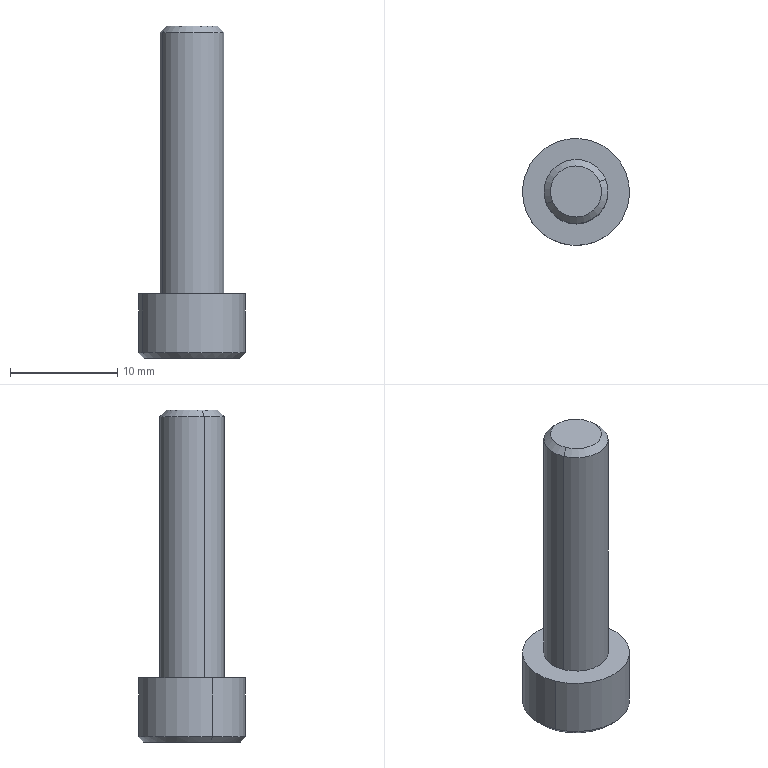Component | SolidWorks | ScrewTAC21-M6-L25(YIHEDA)-5 | 1 solid | 25 faces | box 10 x 10 x 31 mm | volume 1097 mm3 | plane 15 | cone 6 | cylinder 4 | commonest cylinder face diameters 10 x2 6 x2
STEP:
#1=COLOUR_RGB('',0.7922,0.8196,0.9333);
#2=FILL_AREA_STYLE_COLOUR('',#1);
#3=FILL_AREA_STYLE('',(#2));
#4=SURFACE_STYLE_FILL_AREA(#3);
#5=SURFACE_SIDE_STYLE('',(#4));
#6=SURFACE_STYLE_USAGE(.BOTH.,#5);
#7=PRESENTATION_STYLE_ASSIGNMENT((#6));
#8=CARTESIAN_POINT('',(0.3955,1.405,2.949));
#9=VERTEX_POINT('',#8);
#10=CARTESIAN_POINT('',(0.2219,1.333,2.949));
#11=VERTEX_POINT('',#10);
#12=CARTESIAN_POINT('',(0.3087,1.369,2.949));
#13=DIRECTION('',(0.,0.,1.));
#14=DIRECTION('',(0.9237,0.383,0.));
#15=AXIS2_PLACEMENT_3D('',#12,#13,#14);
#16=CIRCLE('',#15,0.09396);
#17=EDGE_CURVE('',#9,#11,#16,.T.);
#18=ORIENTED_EDGE('',*,*,#17,.F.);
#19=CARTESIAN_POINT('',(0.4178,1.414,2.925));
#20=VERTEX_POINT('',#19);
#21=CARTESIAN_POINT('',(0.4178,1.414,2.925));
#22=DIRECTION('',(0.6532,0.2709,-0.7071));
#23=VECTOR('',#22,39.37);
#24=LINE('',#21,#23);
#25=EDGE_CURVE('',#9,#20,#24,.T.);
#26=ORIENTED_EDGE('',*,*,#25,.T.);
#27=CARTESIAN_POINT('',(0.1996,1.323,2.925));
#28=VERTEX_POINT('',#27);
#29=CARTESIAN_POINT('',(0.3087,1.369,2.925));
#30=DIRECTION('',(0.,0.,1.));
#31=DIRECTION('',(0.9237,0.383,0.));
#32=AXIS2_PLACEMENT_3D('',#29,#30,#31);
#33=CIRCLE('',#32,0.1181);
#34=EDGE_CURVE('',#20,#28,#33,.T.);
#35=ORIENTED_EDGE('',*,*,#34,.T.);
#36=CARTESIAN_POINT('',(0.1996,1.323,2.925));
#37=DIRECTION('',(-0.6532,-0.2709,-0.7071));
#38=VECTOR('',#37,39.37);
#39=LINE('',#36,#38);
#40=EDGE_CURVE('',#11,#28,#39,.T.);
#41=ORIENTED_EDGE('',*,*,#40,.F.);
#42=EDGE_LOOP('',(#18,#26,#35,#41));
#43=FACE_OUTER_BOUND('',#42,.T.);
#44=CARTESIAN_POINT('',(0.3087,1.369,2.925));
#45=DIRECTION('',(0.,0.,-1.));
#46=DIRECTION('',(-0.9237,-0.383,0.));
#47=AXIS2_PLACEMENT_3D('',#44,#45,#46);
#48=CONICAL_SURFACE('',#47,0.1181,0.7854);
#49=ADVANCED_FACE('',(#43),#48,.T.);
#50=CARTESIAN_POINT('',(0.4723,1.437,1.728));
#51=VERTEX_POINT('',#50);
#52=CARTESIAN_POINT('',(0.145,1.301,1.728));
#53=VERTEX_POINT('',#52);
#54=CARTESIAN_POINT('',(0.3087,1.369,1.728));
#55=DIRECTION('',(0.,0.,1.));
#56=DIRECTION('',(0.9237,0.383,0.));
#57=AXIS2_PLACEMENT_3D('',#54,#55,#56);
#58=CIRCLE('',#57,0.1772);
#59=EDGE_CURVE('',#51,#53,#58,.T.);
#60=ORIENTED_EDGE('',*,*,#59,.T.);
#61=CARTESIAN_POINT('',(0.1268,1.293,1.748));
#62=VERTEX_POINT('',#61);
#63=CARTESIAN_POINT('',(0.145,1.301,1.728));
#64=DIRECTION('',(-0.6532,-0.2709,0.7071));
#65=VECTOR('',#64,39.37);
#66=LINE('',#63,#65);
#67=EDGE_CURVE('',#53,#62,#66,.T.);
#68=ORIENTED_EDGE('',*,*,#67,.T.);
#69=CARTESIAN_POINT('',(0.4905,1.444,1.748));
#70=VERTEX_POINT('',#69);
#71=CARTESIAN_POINT('',(0.3087,1.369,1.748));
#72=DIRECTION('',(0.,0.,1.));
#73=DIRECTION('',(0.9237,0.383,0.));
#74=AXIS2_PLACEMENT_3D('',#71,#72,#73);
#75=CIRCLE('',#74,0.1969);
#76=EDGE_CURVE('',#70,#62,#75,.T.);
#77=ORIENTED_EDGE('',*,*,#76,.F.);
#78=CARTESIAN_POINT('',(0.4723,1.437,1.728));
#79=DIRECTION('',(0.6532,0.2709,0.7071));
#80=VECTOR('',#79,39.37);
#81=LINE('',#78,#80);
#82=EDGE_CURVE('',#51,#70,#81,.T.);
#83=ORIENTED_EDGE('',*,*,#82,.F.);
#84=EDGE_LOOP('',(#60,#68,#77,#83));
#85=FACE_OUTER_BOUND('',#84,.T.);
#86=CARTESIAN_POINT('',(0.3087,1.369,1.728));
#87=DIRECTION('',(0.,0.,1.));
#88=DIRECTION('',(0.9237,0.383,0.));
#89=AXIS2_PLACEMENT_3D('',#86,#87,#88);
#90=CONICAL_SURFACE('',#89,0.1772,0.7854);
#91=ADVANCED_FACE('',(#85),#90,.T.);
#92=CARTESIAN_POINT('',(0.1268,1.293,1.965));
#93=VERTEX_POINT('',#92);
#94=CARTESIAN_POINT('',(0.4905,1.444,1.965));
#95=VERTEX_POINT('',#94);
#96=CARTESIAN_POINT('',(0.3087,1.369,1.965));
#97=DIRECTION('',(0.,0.,1.));
#98=DIRECTION('',(0.9237,0.383,0.));
#99=AXIS2_PLACEMENT_3D('',#96,#97,#98);
#100=CIRCLE('',#99,0.1969);
#101=EDGE_CURVE('',#93,#95,#100,.T.);
#102=ORIENTED_EDGE('',*,*,#101,.F.);
#103=CARTESIAN_POINT('',(0.1268,1.293,1.965));
#104=DIRECTION('',(0.,0.,-1.));
#105=VECTOR('',#104,39.37);
#106=LINE('',#103,#105);
#107=EDGE_CURVE('',#93,#62,#106,.T.);
#108=ORIENTED_EDGE('',*,*,#107,.T.);
#109=CARTESIAN_POINT('',(0.3087,1.369,1.748));
#110=DIRECTION('',(0.,0.,1.));
#111=DIRECTION('',(0.9237,0.383,0.));
#112=AXIS2_PLACEMENT_3D('',#109,#110,#111);
#113=CIRCLE('',#112,0.1969);
#114=EDGE_CURVE('',#62,#70,#113,.T.);
#115=ORIENTED_EDGE('',*,*,#114,.T.);
#116=CARTESIAN_POINT('',(0.4905,1.444,1.965));
#117=DIRECTION('',(0.,0.,-1.));
#118=VECTOR('',#117,39.37);
#119=LINE('',#116,#118);
#120=EDGE_CURVE('',#95,#70,#119,.T.);
#121=ORIENTED_EDGE('',*,*,#120,.F.);
#122=EDGE_LOOP('',(#102,#108,#115,#121));
#123=FACE_OUTER_BOUND('',#122,.T.);
#124=CARTESIAN_POINT('',(0.3087,1.369,1.965));
#125=DIRECTION('',(0.,0.,-1.));
#126=DIRECTION('',(0.9237,0.383,0.));
#127=AXIS2_PLACEMENT_3D('',#124,#125,#126);
#128=CYLINDRICAL_SURFACE('',#127,0.1969);
#129=ADVANCED_FACE('',(#123),#128,.T.);
#130=CARTESIAN_POINT('',(0.3087,1.369,1.903));
#131=VERTEX_POINT('',#130);
#132=CARTESIAN_POINT('',(0.2178,1.331,1.847));
#133=VERTEX_POINT('',#132);
#134=CARTESIAN_POINT('',(0.2178,1.331,1.847));
#135=DIRECTION('',(-0.8,-0.3317,-0.5));
#136=VECTOR('',#135,39.37);
#137=LINE('',#134,#136);
#138=EDGE_CURVE('',#131,#133,#137,.T.);
#139=ORIENTED_EDGE('',*,*,#138,.F.);
#140=CARTESIAN_POINT('',(0.3996,1.406,1.847));
#141=VERTEX_POINT('',#140);
#142=CARTESIAN_POINT('',(0.3996,1.406,1.847));
#143=DIRECTION('',(0.8,0.3317,-0.5));
#144=VECTOR('',#143,39.37);
#145=LINE('',#142,#144);
#146=EDGE_CURVE('',#131,#141,#145,.T.);
#147=ORIENTED_EDGE('',*,*,#146,.T.);
#148=CARTESIAN_POINT('',(0.3868,1.309,1.847));
#149=VERTEX_POINT('',#148);
#150=CARTESIAN_POINT('',(0.3087,1.369,1.847));
#151=DIRECTION('',(0.,0.,1.));
#152=DIRECTION('',(-0.9237,-0.383,0.));
#153=AXIS2_PLACEMENT_3D('',#150,#151,#152);
#154=CIRCLE('',#153,0.09843);
#155=EDGE_CURVE('',#149,#141,#154,.T.);
#156=ORIENTED_EDGE('',*,*,#155,.F.);
#157=CARTESIAN_POINT('',(0.2959,1.271,1.847));
#158=VERTEX_POINT('',#157);
#159=CARTESIAN_POINT('',(0.3087,1.369,1.847));
#160=DIRECTION('',(0.,0.,1.));
#161=DIRECTION('',(-0.9237,-0.383,0.));
#162=AXIS2_PLACEMENT_3D('',#159,#160,#161);
#163=CIRCLE('',#162,0.09843);
#164=EDGE_CURVE('',#158,#149,#163,.T.);
#165=ORIENTED_EDGE('',*,*,#164,.F.);
#166=CARTESIAN_POINT('',(0.3087,1.369,1.847));
#167=DIRECTION('',(0.,0.,1.));
#168=DIRECTION('',(-0.9237,-0.383,0.));
#169=AXIS2_PLACEMENT_3D('',#166,#167,#168);
#170=CIRCLE('',#169,0.09843);
#171=EDGE_CURVE('',#133,#158,#170,.T.);
#172=ORIENTED_EDGE('',*,*,#171,.F.);
#173=EDGE_LOOP('',(#139,#147,#156,#165,#172));
#174=FACE_OUTER_BOUND('',#173,.T.);
#175=CARTESIAN_POINT('',(0.3087,1.369,1.847));
#176=DIRECTION('',(0.,0.,-1.));
#177=DIRECTION('',(-0.9237,-0.383,0.));
#178=AXIS2_PLACEMENT_3D('',#175,#176,#177);
#179=CONICAL_SURFACE('',#178,0.09843,1.047);
#180=ADVANCED_FACE('',(#174),#179,.F.);
#181=CARTESIAN_POINT('',(0.3087,1.369,2.925));
#182=DIRECTION('',(0.,0.,1.));
#183=DIRECTION('',(0.9237,0.383,0.));
#184=AXIS2_PLACEMENT_3D('',#181,#182,#183);
#185=CIRCLE('',#184,0.1181);
#186=EDGE_CURVE('',#28,#20,#185,.T.);
#187=ORIENTED_EDGE('',*,*,#186,.F.);
#188=CARTESIAN_POINT('',(0.1996,1.323,1.965));
#189=VERTEX_POINT('',#188);
#190=CARTESIAN_POINT('',(0.1996,1.323,2.949));
#191=DIRECTION('',(0.,0.,-1.));
#192=VECTOR('',#191,39.37);
#193=LINE('',#190,#192);
#194=EDGE_CURVE('',#28,#189,#193,.T.);
#195=ORIENTED_EDGE('',*,*,#194,.T.);
#196=CARTESIAN_POINT('',(0.4178,1.414,1.965));
#197=VERTEX_POINT('',#196);
#198=CARTESIAN_POINT('',(0.3087,1.369,1.965));
#199=DIRECTION('',(0.,0.,1.));
#200=DIRECTION('',(0.9237,0.383,0.));
#201=AXIS2_PLACEMENT_3D('',#198,#199,#200);
#202=CIRCLE('',#201,0.1181);
#203=EDGE_CURVE('',#189,#197,#202,.T.);
#204=ORIENTED_EDGE('',*,*,#203,.T.);
#205=CARTESIAN_POINT('',(0.4178,1.414,2.949));
#206=DIRECTION('',(0.,0.,-1.));
#207=VECTOR('',#206,39.37);
#208=LINE('',#205,#207);
#209=EDGE_CURVE('',#20,#197,#208,.T.);
#210=ORIENTED_EDGE('',*,*,#209,.F.);
#211=EDGE_LOOP('',(#187,#195,#204,#210));
#212=FACE_OUTER_BOUND('',#211,.T.);
#213=CARTESIAN_POINT('',(0.3087,1.369,2.949));
#214=DIRECTION('',(0.,0.,-1.));
#215=DIRECTION('',(0.9237,0.383,0.));
#216=AXIS2_PLACEMENT_3D('',#213,#214,#215);
#217=CYLINDRICAL_SURFACE('',#216,0.1181);
#218=ADVANCED_FACE('',(#212),#217,.T.);
#219=CARTESIAN_POINT('',(0.3522,1.264,1.847));
#220=VERTEX_POINT('',#219);
#221=CARTESIAN_POINT('',(0.3522,1.264,1.847));
#222=DIRECTION('',(-0.9915,0.1301,0.));
#223=VECTOR('',#222,39.37);
#224=LINE('',#221,#223);
#225=EDGE_CURVE('',#220,#158,#224,.T.);
#226=ORIENTED_EDGE('',*,*,#225,.T.);
#227=ORIENTED_EDGE('',*,*,#164,.T.);
#228=CARTESIAN_POINT('',(0.4214,1.354,1.847));
#229=DIRECTION('',(-0.6084,-0.7936,0.));
#230=VECTOR('',#229,39.37);
#231=LINE('',#228,#230);
#232=EDGE_CURVE('',#149,#220,#231,.T.);
#233=ORIENTED_EDGE('',*,*,#232,.T.);
#234=EDGE_LOOP('',(#226,#227,#233));
#235=FACE_OUTER_BOUND('',#234,.T.);
#236=CARTESIAN_POINT('',(0.3087,1.369,1.847));
#237=DIRECTION('',(0.,0.,-1.));
#238=DIRECTION('',(-0.9237,-0.383,0.));
#239=AXIS2_PLACEMENT_3D('',#236,#237,#238);
#240=PLANE('',#239);
#241=ADVANCED_FACE('',(#235),#240,.T.);
#242=ORIENTED_EDGE('',*,*,#194,.F.);
#243=ORIENTED_EDGE('',*,*,#34,.F.);
#244=ORIENTED_EDGE('',*,*,#209,.T.);
#245=CARTESIAN_POINT('',(0.3087,1.369,1.965));
#246=DIRECTION('',(0.,0.,1.));
#247=DIRECTION('',(0.9237,0.383,0.));
#248=AXIS2_PLACEMENT_3D('',#245,#246,#247);
#249=CIRCLE('',#248,0.1181);
#250=EDGE_CURVE('',#197,#189,#249,.T.);
#251=ORIENTED_EDGE('',*,*,#250,.T.);
#252=EDGE_LOOP('',(#242,#243,#244,#251));
#253=FACE_OUTER_BOUND('',#252,.T.);
#254=CARTESIAN_POINT('',(0.3087,1.369,2.949));
#255=DIRECTION('',(0.,0.,-1.));
#256=DIRECTION('',(0.9237,0.383,0.));
#257=AXIS2_PLACEMENT_3D('',#254,#255,#256);
#258=CYLINDRICAL_SURFACE('',#257,0.1181);
#259=ADVANCED_FACE('',(#253),#258,.T.);
#260=ORIENTED_EDGE('',*,*,#146,.F.);
#261=ORIENTED_EDGE('',*,*,#138,.T.);
#262=CARTESIAN_POINT('',(0.2306,1.429,1.847));
#263=VERTEX_POINT('',#262);
#264=CARTESIAN_POINT('',(0.3087,1.369,1.847));
#265=DIRECTION('',(0.,0.,1.));
#266=DIRECTION('',(-0.9237,-0.383,0.));
#267=AXIS2_PLACEMENT_3D('',#264,#265,#266);
#268=CIRCLE('',#267,0.09843);
#269=EDGE_CURVE('',#263,#133,#268,.T.);
#270=ORIENTED_EDGE('',*,*,#269,.F.);
#271=CARTESIAN_POINT('',(0.3215,1.466,1.847));
#272=VERTEX_POINT('',#271);
#273=CARTESIAN_POINT('',(0.3087,1.369,1.847));
#274=DIRECTION('',(0.,0.,1.));
#275=DIRECTION('',(-0.9237,-0.383,0.));
#276=AXIS2_PLACEMENT_3D('',#273,#274,#275);
#277=CIRCLE('',#276,0.09843);
#278=EDGE_CURVE('',#272,#263,#277,.T.);
#279=ORIENTED_EDGE('',*,*,#278,.F.);
#280=CARTESIAN_POINT('',(0.3087,1.369,1.847));
#281=DIRECTION('',(0.,0.,1.));
#282=DIRECTION('',(-0.9237,-0.383,0.));
#283=AXIS2_PLACEMENT_3D('',#280,#281,#282);
#284=CIRCLE('',#283,0.09843);
#285=EDGE_CURVE('',#141,#272,#284,.T.);
#286=ORIENTED_EDGE('',*,*,#285,.F.);
#287=EDGE_LOOP('',(#260,#261,#270,#279,#286));
#288=FACE_OUTER_BOUND('',#287,.T.);
#289=CARTESIAN_POINT('',(0.3087,1.369,1.847));
#290=DIRECTION('',(0.,0.,-1.));
#291=DIRECTION('',(-0.9237,-0.383,0.));
#292=AXIS2_PLACEMENT_3D('',#289,#290,#291);
#293=CONICAL_SURFACE('',#292,0.09843,1.047);
#294=ADVANCED_FACE('',(#288),#293,.F.);
#295=CARTESIAN_POINT('',(0.3778,1.459,1.728));
#296=VERTEX_POINT('',#295);
#297=CARTESIAN_POINT('',(0.4214,1.354,1.728));
#298=VERTEX_POINT('',#297);
#299=CARTESIAN_POINT('',(0.3778,1.459,1.728));
#300=DIRECTION('',(0.383,-0.9237,0.));
#301=VECTOR('',#300,39.37);
#302=LINE('',#299,#301);
#303=EDGE_CURVE('',#296,#298,#302,.T.);
#304=ORIENTED_EDGE('',*,*,#303,.T.);
#305=CARTESIAN_POINT('',(0.4214,1.354,1.847));
#306=VERTEX_POINT('',#305);
#307=CARTESIAN_POINT('',(0.4214,1.354,1.847));
#308=DIRECTION('',(0.,0.,-1.));
#309=VECTOR('',#308,39.37);
#310=LINE('',#307,#309);
#311=EDGE_CURVE('',#306,#298,#310,.T.);
#312=ORIENTED_EDGE('',*,*,#311,.F.);
#313=CARTESIAN_POINT('',(0.3778,1.459,1.847));
#314=DIRECTION('',(0.383,-0.9237,0.));
#315=VECTOR('',#314,39.37);
#316=LINE('',#313,#315);
#317=EDGE_CURVE('',#141,#306,#316,.T.);
#318=ORIENTED_EDGE('',*,*,#317,.F.);
#319=CARTESIAN_POINT('',(0.3778,1.459,1.847));
#320=VERTEX_POINT('',#319);
#321=CARTESIAN_POINT('',(0.3778,1.459,1.847));
#322=DIRECTION('',(0.383,-0.9237,0.));
#323=VECTOR('',#322,39.37);
#324=LINE('',#321,#323);
#325=EDGE_CURVE('',#320,#141,#324,.T.);
#326=ORIENTED_EDGE('',*,*,#325,.F.);
#327=CARTESIAN_POINT('',(0.3778,1.459,1.847));
#328=DIRECTION('',(0.,0.,-1.));
#329=VECTOR('',#328,39.37);
#330=LINE('',#327,#329);
#331=EDGE_CURVE('',#320,#296,#330,.T.);
#332=ORIENTED_EDGE('',*,*,#331,.T.);
#333=EDGE_LOOP('',(#304,#312,#318,#326,#332));
#334=FACE_OUTER_BOUND('',#333,.T.);
#335=CARTESIAN_POINT('',(0.3778,1.459,1.847));
#336=DIRECTION('',(0.9237,0.383,0.));
#337=DIRECTION('',(0.,0.,-1.));
#338=AXIS2_PLACEMENT_3D('',#335,#336,#337);
#339=PLANE('',#338);
#340=ADVANCED_FACE('',(#334),#339,.F.);
#341=CARTESIAN_POINT('',(0.196,1.384,1.728));
#342=VERTEX_POINT('',#341);
#343=CARTESIAN_POINT('',(0.2651,1.474,1.728));
#344=VERTEX_POINT('',#343);
#345=CARTESIAN_POINT('',(0.196,1.384,1.728));
#346=DIRECTION('',(0.6084,0.7936,0.));
#347=VECTOR('',#346,39.37);
#348=LINE('',#345,#347);
#349=EDGE_CURVE('',#342,#344,#348,.T.);
#350=ORIENTED_EDGE('',*,*,#349,.T.);
#351=CARTESIAN_POINT('',(0.2651,1.474,1.847));
#352=VERTEX_POINT('',#351);
#353=CARTESIAN_POINT('',(0.2651,1.474,1.847));
#354=DIRECTION('',(0.,0.,-1.));
#355=VECTOR('',#354,39.37);
#356=LINE('',#353,#355);
#357=EDGE_CURVE('',#352,#344,#356,.T.);
#358=ORIENTED_EDGE('',*,*,#357,.F.);
#359=CARTESIAN_POINT('',(0.196,1.384,1.847));
#360=DIRECTION('',(0.6084,0.7936,0.));
#361=VECTOR('',#360,39.37);
#362=LINE('',#359,#361);
#363=EDGE_CURVE('',#263,#352,#362,.T.);
#364=ORIENTED_EDGE('',*,*,#363,.F.);
#365=CARTESIAN_POINT('',(0.196,1.384,1.847));
#366=VERTEX_POINT('',#365);
#367=CARTESIAN_POINT('',(0.196,1.384,1.847));
#368=DIRECTION('',(0.6084,0.7936,0.));
#369=VECTOR('',#368,39.37);
#370=LINE('',#367,#369);
#371=EDGE_CURVE('',#366,#263,#370,.T.);
#372=ORIENTED_EDGE('',*,*,#371,.F.);
#373=CARTESIAN_POINT('',(0.196,1.384,1.847));
#374=DIRECTION('',(0.,0.,-1.));
#375=VECTOR('',#374,39.37);
#376=LINE('',#373,#375);
#377=EDGE_CURVE('',#366,#342,#376,.T.);
#378=ORIENTED_EDGE('',*,*,#377,.T.);
#379=EDGE_LOOP('',(#350,#358,#364,#372,#378));
#380=FACE_OUTER_BOUND('',#379,.T.);
#381=CARTESIAN_POINT('',(0.196,1.384,1.847));
#382=DIRECTION('',(-0.7936,0.6084,0.));
#383=DIRECTION('',(0.,0.,1.));
#384=AXIS2_PLACEMENT_3D('',#381,#382,#383);
#385=PLANE('',#384);
#386=ADVANCED_FACE('',(#380),#385,.F.);
#387=ORIENTED_EDGE('',*,*,#371,.T.);
#388=ORIENTED_EDGE('',*,*,#269,.T.);
#389=CARTESIAN_POINT('',(0.2395,1.279,1.847));
#390=DIRECTION('',(-0.383,0.9237,0.));
#391=VECTOR('',#390,39.37);
#392=LINE('',#389,#391);
#393=EDGE_CURVE('',#133,#366,#392,.T.);
#394=ORIENTED_EDGE('',*,*,#393,.T.);
#395=EDGE_LOOP('',(#387,#388,#394));
#396=FACE_OUTER_BOUND('',#395,.T.);
#397=CARTESIAN_POINT('',(0.3087,1.369,1.847));
#398=DIRECTION('',(0.,0.,-1.));
#399=DIRECTION('',(-0.9237,-0.383,0.));
#400=AXIS2_PLACEMENT_3D('',#397,#398,#399);
#401=PLANE('',#400);
#402=ADVANCED_FACE('',(#396),#401,.T.);
#403=CARTESIAN_POINT('',(0.3087,1.369,1.965));
#404=DIRECTION('',(0.,0.,1.));
#405=DIRECTION('',(0.9237,0.383,0.));
#406=AXIS2_PLACEMENT_3D('',#403,#404,#405);
#407=CIRCLE('',#406,0.1969);
#408=EDGE_CURVE('',#95,#93,#407,.T.);
#409=ORIENTED_EDGE('',*,*,#408,.T.);
#410=ORIENTED_EDGE('',*,*,#101,.T.);
#411=EDGE_LOOP('',(#409,#410));
#412=FACE_OUTER_BOUND('',#411,.T.);
#413=ORIENTED_EDGE('',*,*,#250,.F.);
#414=ORIENTED_EDGE('',*,*,#203,.F.);
#415=EDGE_LOOP('',(#413,#414));
#416=FACE_BOUND('',#415,.T.);
#417=CARTESIAN_POINT('',(0.2333,1.551,1.965));
#418=DIRECTION('',(0.,0.,-1.));
#419=DIRECTION('',(-0.9237,-0.383,0.));
#420=AXIS2_PLACEMENT_3D('',#417,#418,#419);
#421=PLANE('',#420);
#422=ADVANCED_FACE('',(#412,#416),#421,.F.);
#423=ORIENTED_EDGE('',*,*,#59,.F.);
#424=CARTESIAN_POINT('',(0.3087,1.369,1.728));
#425=DIRECTION('',(0.,0.,1.));
#426=DIRECTION('',(0.9237,0.383,0.));
#427=AXIS2_PLACEMENT_3D('',#424,#425,#426);
#428=CIRCLE('',#427,0.1772);
#429=EDGE_CURVE('',#53,#51,#428,.T.);
#430=ORIENTED_EDGE('',*,*,#429,.F.);
#431=EDGE_LOOP('',(#423,#430));
#432=FACE_OUTER_BOUND('',#431,.T.);
#433=CARTESIAN_POINT('',(0.3522,1.264,1.728));
#434=VERTEX_POINT('',#433);
#435=CARTESIAN_POINT('',(0.2395,1.279,1.728));
#436=VERTEX_POINT('',#435);
#437=CARTESIAN_POINT('',(0.3522,1.264,1.728));
#438=DIRECTION('',(-0.9915,0.1301,0.));
#439=VECTOR('',#438,39.37);
#440=LINE('',#437,#439);
#441=EDGE_CURVE('',#434,#436,#440,.T.);
#442=ORIENTED_EDGE('',*,*,#441,.F.);
#443=CARTESIAN_POINT('',(0.4214,1.354,1.728));
#444=DIRECTION('',(-0.6084,-0.7936,0.));
#445=VECTOR('',#444,39.37);
#446=LINE('',#443,#445);
#447=EDGE_CURVE('',#298,#434,#446,.T.);
#448=ORIENTED_EDGE('',*,*,#447,.F.);
#449=ORIENTED_EDGE('',*,*,#303,.F.);
#450=CARTESIAN_POINT('',(0.2651,1.474,1.728));
#451=DIRECTION('',(0.9915,-0.1301,0.));
#452=VECTOR('',#451,39.37);
#453=LINE('',#450,#452);
#454=EDGE_CURVE('',#344,#296,#453,.T.);
#455=ORIENTED_EDGE('',*,*,#454,.F.);
#456=ORIENTED_EDGE('',*,*,#349,.F.);
#457=CARTESIAN_POINT('',(0.2395,1.279,1.728));
#458=DIRECTION('',(-0.383,0.9237,0.));
#459=VECTOR('',#458,39.37);
#460=LINE('',#457,#459);
#461=EDGE_CURVE('',#436,#342,#460,.T.);
#462=ORIENTED_EDGE('',*,*,#461,.F.);
#463=EDGE_LOOP('',(#442,#448,#449,#455,#456,#462));
#464=FACE_BOUND('',#463,.T.);
#465=CARTESIAN_POINT('',(0.3087,1.369,1.728));
#466=DIRECTION('',(0.,0.,1.));
#467=DIRECTION('',(0.383,-0.9237,0.));
#468=AXIS2_PLACEMENT_3D('',#465,#466,#467);
#469=PLANE('',#468);
#470=ADVANCED_FACE('',(#432,#464),#469,.F.);
#471=CARTESIAN_POINT('',(0.3087,1.369,2.949));
#472=DIRECTION('',(0.,0.,1.));
#473=DIRECTION('',(0.9237,0.383,0.));
#474=AXIS2_PLACEMENT_3D('',#471,#472,#473);
#475=CIRCLE('',#474,0.09396);
#476=EDGE_CURVE('',#11,#9,#475,.T.);
#477=ORIENTED_EDGE('',*,*,#476,.T.);
#478=ORIENTED_EDGE('',*,*,#17,.T.);
#479=EDGE_LOOP('',(#477,#478));
#480=FACE_OUTER_BOUND('',#479,.T.);
#481=CARTESIAN_POINT('',(0.2727,1.456,2.949));
#482=DIRECTION('',(0.,0.,-1.));
#483=DIRECTION('',(-0.9237,-0.383,0.));
#484=AXIS2_PLACEMENT_3D('',#481,#482,#483);
#485=PLANE('',#484);
#486=ADVANCED_FACE('',(#480),#485,.F.);
#487=ORIENTED_EDGE('',*,*,#107,.F.);
#488=ORIENTED_EDGE('',*,*,#408,.F.);
#489=ORIENTED_EDGE('',*,*,#120,.T.);
#490=ORIENTED_EDGE('',*,*,#76,.T.);
#491=EDGE_LOOP('',(#487,#488,#489,#490));
#492=FACE_OUTER_BOUND('',#491,.T.);
#493=CARTESIAN_POINT('',(0.3087,1.369,1.965));
#494=DIRECTION('',(0.,0.,-1.));
#495=DIRECTION('',(0.9237,0.383,0.));
#496=AXIS2_PLACEMENT_3D('',#493,#494,#495);
#497=CYLINDRICAL_SURFACE('',#496,0.1969);
#498=ADVANCED_FACE('',(#492),#497,.T.);
#499=ORIENTED_EDGE('',*,*,#447,.T.);
#500=CARTESIAN_POINT('',(0.3522,1.264,1.847));
#501=DIRECTION('',(0.,0.,-1.));
#502=VECTOR('',#501,39.37);
#503=LINE('',#500,#502);
#504=EDGE_CURVE('',#220,#434,#503,.T.);
#505=ORIENTED_EDGE('',*,*,#504,.F.);
#506=ORIENTED_EDGE('',*,*,#232,.F.);
#507=CARTESIAN_POINT('',(0.4214,1.354,1.847));
#508=DIRECTION('',(-0.6084,-0.7936,0.));
#509=VECTOR('',#508,39.37);
#510=LINE('',#507,#509);
#511=EDGE_CURVE('',#306,#149,#510,.T.);
#512=ORIENTED_EDGE('',*,*,#511,.F.);
#513=ORIENTED_EDGE('',*,*,#311,.T.);
#514=EDGE_LOOP('',(#499,#505,#506,#512,#513));
#515=FACE_OUTER_BOUND('',#514,.T.);
#516=CARTESIAN_POINT('',(0.4214,1.354,1.847));
#517=DIRECTION('',(0.7936,-0.6084,0.));
#518=DIRECTION('',(0.6084,0.7936,0.));
#519=AXIS2_PLACEMENT_3D('',#516,#517,#518);
#520=PLANE('',#519);
#521=ADVANCED_FACE('',(#515),#520,.F.);
#522=ORIENTED_EDGE('',*,*,#67,.F.);
#523=ORIENTED_EDGE('',*,*,#429,.T.);
#524=ORIENTED_EDGE('',*,*,#82,.T.);
#525=ORIENTED_EDGE('',*,*,#114,.F.);
#526=EDGE_LOOP('',(#522,#523,#524,#525));
#527=FACE_OUTER_BOUND('',#526,.T.);
#528=CARTESIAN_POINT('',(0.3087,1.369,1.728));
#529=DIRECTION('',(0.,0.,1.));
#530=DIRECTION('',(0.9237,0.383,0.));
#531=AXIS2_PLACEMENT_3D('',#528,#529,#530);
#532=CONICAL_SURFACE('',#531,0.1772,0.7854);
#533=ADVANCED_FACE('',(#527),#532,.T.);
#534=ORIENTED_EDGE('',*,*,#441,.T.);
#535=CARTESIAN_POINT('',(0.2395,1.279,1.847));
#536=VERTEX_POINT('',#535);
#537=CARTESIAN_POINT('',(0.2395,1.279,1.847));
#538=DIRECTION('',(0.,0.,-1.));
#539=VECTOR('',#538,39.37);
#540=LINE('',#537,#539);
#541=EDGE_CURVE('',#536,#436,#540,.T.);
#542=ORIENTED_EDGE('',*,*,#541,.F.);
#543=CARTESIAN_POINT('',(0.3522,1.264,1.847));
#544=DIRECTION('',(-0.9915,0.1301,0.));
#545=VECTOR('',#544,39.37);
#546=LINE('',#543,#545);
#547=EDGE_CURVE('',#158,#536,#546,.T.);
#548=ORIENTED_EDGE('',*,*,#547,.F.);
#549=ORIENTED_EDGE('',*,*,#225,.F.);
#550=ORIENTED_EDGE('',*,*,#504,.T.);
#551=EDGE_LOOP('',(#534,#542,#548,#549,#550));
#552=FACE_OUTER_BOUND('',#551,.T.);
#553=CARTESIAN_POINT('',(0.3522,1.264,1.847));
#554=DIRECTION('',(-0.1301,-0.9915,0.));
#555=DIRECTION('',(0.,0.,1.));
#556=AXIS2_PLACEMENT_3D('',#553,#554,#555);
#557=PLANE('',#556);
#558=ADVANCED_FACE('',(#552),#557,.F.);
#559=ORIENTED_EDGE('',*,*,#461,.T.);
#560=ORIENTED_EDGE('',*,*,#377,.F.);
#561=ORIENTED_EDGE('',*,*,#393,.F.);
#562=CARTESIAN_POINT('',(0.2395,1.279,1.847));
#563=DIRECTION('',(-0.383,0.9237,0.));
#564=VECTOR('',#563,39.37);
#565=LINE('',#562,#564);
#566=EDGE_CURVE('',#536,#133,#565,.T.);
#567=ORIENTED_EDGE('',*,*,#566,.F.);
#568=ORIENTED_EDGE('',*,*,#541,.T.);
#569=EDGE_LOOP('',(#559,#560,#561,#567,#568));
#570=FACE_OUTER_BOUND('',#569,.T.);
#571=CARTESIAN_POINT('',(0.2395,1.279,1.847));
#572=DIRECTION('',(-0.9237,-0.383,0.));
#573=DIRECTION('',(-0.383,0.9237,0.));
#574=AXIS2_PLACEMENT_3D('',#571,#572,#573);
#575=PLANE('',#574);
#576=ADVANCED_FACE('',(#570),#575,.F.);
#577=ORIENTED_EDGE('',*,*,#566,.T.);
#578=ORIENTED_EDGE('',*,*,#171,.T.);
#579=ORIENTED_EDGE('',*,*,#547,.T.);
#580=EDGE_LOOP('',(#577,#578,#579));
#581=FACE_OUTER_BOUND('',#580,.T.);
#582=CARTESIAN_POINT('',(0.3087,1.369,1.847));
#583=DIRECTION('',(0.,0.,-1.));
#584=DIRECTION('',(-0.9237,-0.383,0.));
#585=AXIS2_PLACEMENT_3D('',#582,#583,#584);
#586=PLANE('',#585);
#587=ADVANCED_FACE('',(#581),#586,.T.);
#588=ORIENTED_EDGE('',*,*,#511,.T.);
#589=ORIENTED_EDGE('',*,*,#155,.T.);
#590=ORIENTED_EDGE('',*,*,#317,.T.);
#591=EDGE_LOOP('',(#588,#589,#590));
#592=FACE_OUTER_BOUND('',#591,.T.);
#593=CARTESIAN_POINT('',(0.3087,1.369,1.847));
#594=DIRECTION('',(0.,0.,-1.));
#595=DIRECTION('',(-0.9237,-0.383,0.));
#596=AXIS2_PLACEMENT_3D('',#593,#594,#595);
#597=PLANE('',#596);
#598=ADVANCED_FACE('',(#592),#597,.T.);
#599=ORIENTED_EDGE('',*,*,#325,.T.);
#600=ORIENTED_EDGE('',*,*,#285,.T.);
#601=CARTESIAN_POINT('',(0.2651,1.474,1.847));
#602=DIRECTION('',(0.9915,-0.1301,0.));
#603=VECTOR('',#602,39.37);
#604=LINE('',#601,#603);
#605=EDGE_CURVE('',#272,#320,#604,.T.);
#606=ORIENTED_EDGE('',*,*,#605,.T.);
#607=EDGE_LOOP('',(#599,#600,#606));
#608=FACE_OUTER_BOUND('',#607,.T.);
#609=CARTESIAN_POINT('',(0.3087,1.369,1.847));
#610=DIRECTION('',(0.,0.,-1.));
#611=DIRECTION('',(-0.9237,-0.383,0.));
#612=AXIS2_PLACEMENT_3D('',#609,#610,#611);
#613=PLANE('',#612);
#614=ADVANCED_FACE('',(#608),#613,.T.);
#615=ORIENTED_EDGE('',*,*,#454,.T.);
#616=ORIENTED_EDGE('',*,*,#331,.F.);
#617=ORIENTED_EDGE('',*,*,#605,.F.);
#618=CARTESIAN_POINT('',(0.2651,1.474,1.847));
#619=DIRECTION('',(0.9915,-0.1301,0.));
#620=VECTOR('',#619,39.37);
#621=LINE('',#618,#620);
#622=EDGE_CURVE('',#352,#272,#621,.T.);
#623=ORIENTED_EDGE('',*,*,#622,.F.);
#624=ORIENTED_EDGE('',*,*,#357,.T.);
#625=EDGE_LOOP('',(#615,#616,#617,#623,#624));
#626=FACE_OUTER_BOUND('',#625,.T.);
#627=CARTESIAN_POINT('',(0.2651,1.474,1.847));
#628=DIRECTION('',(0.1301,0.9915,0.));
#629=DIRECTION('',(0.,0.,-1.));
#630=AXIS2_PLACEMENT_3D('',#627,#628,#629);
#631=PLANE('',#630);
#632=ADVANCED_FACE('',(#626),#631,.F.);
#633=ORIENTED_EDGE('',*,*,#25,.F.);
#634=ORIENTED_EDGE('',*,*,#476,.F.);
#635=ORIENTED_EDGE('',*,*,#40,.T.);
#636=ORIENTED_EDGE('',*,*,#186,.T.);
#637=EDGE_LOOP('',(#633,#634,#635,#636));
#638=FACE_OUTER_BOUND('',#637,.T.);
#639=CARTESIAN_POINT('',(0.3087,1.369,2.925));
#640=DIRECTION('',(0.,0.,-1.));
#641=DIRECTION('',(-0.9237,-0.383,0.));
#642=AXIS2_PLACEMENT_3D('',#639,#640,#641);
#643=CONICAL_SURFACE('',#642,0.1181,0.7854);
#644=ADVANCED_FACE('',(#638),#643,.T.);
#645=ORIENTED_EDGE('',*,*,#622,.T.);
#646=ORIENTED_EDGE('',*,*,#278,.T.);
#647=ORIENTED_EDGE('',*,*,#363,.T.);
#648=EDGE_LOOP('',(#645,#646,#647));
#649=FACE_OUTER_BOUND('',#648,.T.);
#650=CARTESIAN_POINT('',(0.3087,1.369,1.847));
#651=DIRECTION('',(0.,0.,-1.));
#652=DIRECTION('',(-0.9237,-0.383,0.));
#653=AXIS2_PLACEMENT_3D('',#650,#651,#652);
#654=PLANE('',#653);
#655=ADVANCED_FACE('',(#649),#654,.T.);
#656=CLOSED_SHELL('',(#49,#91,#129,#180,#218,#241,#259,#294,#340,#386,#402,#422,#470,#486,#498,#521,#533,#558,#576,#587,#598,#614,#632,#644,#655));
#657=MANIFOLD_SOLID_BREP('',#656);
#658=STYLED_ITEM('',(#7),#657);
#659=PRESENTATION_LAYER_ASSIGNMENT('','',(#658));
#660=(LENGTH_UNIT()NAMED_UNIT(*)SI_UNIT($,.METRE.));
#661=LENGTH_MEASURE_WITH_UNIT(LENGTH_MEASURE(0.0254),#660);
#662=DIMENSIONAL_EXPONENTS(1.,0.,0.,0.,0.,0.,0.);
#663=(CONVERSION_BASED_UNIT('',#661)LENGTH_UNIT()NAMED_UNIT(#662));
#664=UNCERTAINTY_MEASURE_WITH_UNIT(LENGTH_MEASURE(0.00001),#663,'','');
#665=(NAMED_UNIT(*)PLANE_ANGLE_UNIT()SI_UNIT($,.RADIAN.));
#666=(NAMED_UNIT(*)SI_UNIT($,.STERADIAN.)SOLID_ANGLE_UNIT());
#667=(GEOMETRIC_REPRESENTATION_CONTEXT(3)GLOBAL_UNCERTAINTY_ASSIGNED_CONTEXT((#664))GLOBAL_UNIT_ASSIGNED_CONTEXT((#663,#665,#666))REPRESENTATION_CONTEXT('',''));
#668=MECHANICAL_DESIGN_GEOMETRIC_PRESENTATION_REPRESENTATION('',(#658),#667);
#669=CARTESIAN_POINT('',(0.,0.,0.));
#670=DIRECTION('',(0.,0.,1.));
#671=DIRECTION('',(1.,0.,0.));
#672=AXIS2_PLACEMENT_3D('',#669,#670,#671);
#673=(LENGTH_UNIT()NAMED_UNIT(*)SI_UNIT($,.METRE.));
#674=LENGTH_MEASURE_WITH_UNIT(LENGTH_MEASURE(0.0254),#673);
#675=DIMENSIONAL_EXPONENTS(1.,0.,0.,0.,0.,0.,0.);
#676=(CONVERSION_BASED_UNIT('',#674)LENGTH_UNIT()NAMED_UNIT(#675));
#677=UNCERTAINTY_MEASURE_WITH_UNIT(LENGTH_MEASURE(0.00001),#676,'','');
#678=(NAMED_UNIT(*)PLANE_ANGLE_UNIT()SI_UNIT($,.RADIAN.));
#679=(NAMED_UNIT(*)SI_UNIT($,.STERADIAN.)SOLID_ANGLE_UNIT());
#680=(GEOMETRIC_REPRESENTATION_CONTEXT(3)GLOBAL_UNCERTAINTY_ASSIGNED_CONTEXT((#677))GLOBAL_UNIT_ASSIGNED_CONTEXT((#676,#678,#679))REPRESENTATION_CONTEXT('',''));
#681=ADVANCED_BREP_SHAPE_REPRESENTATION('',(#657,#672),#680);